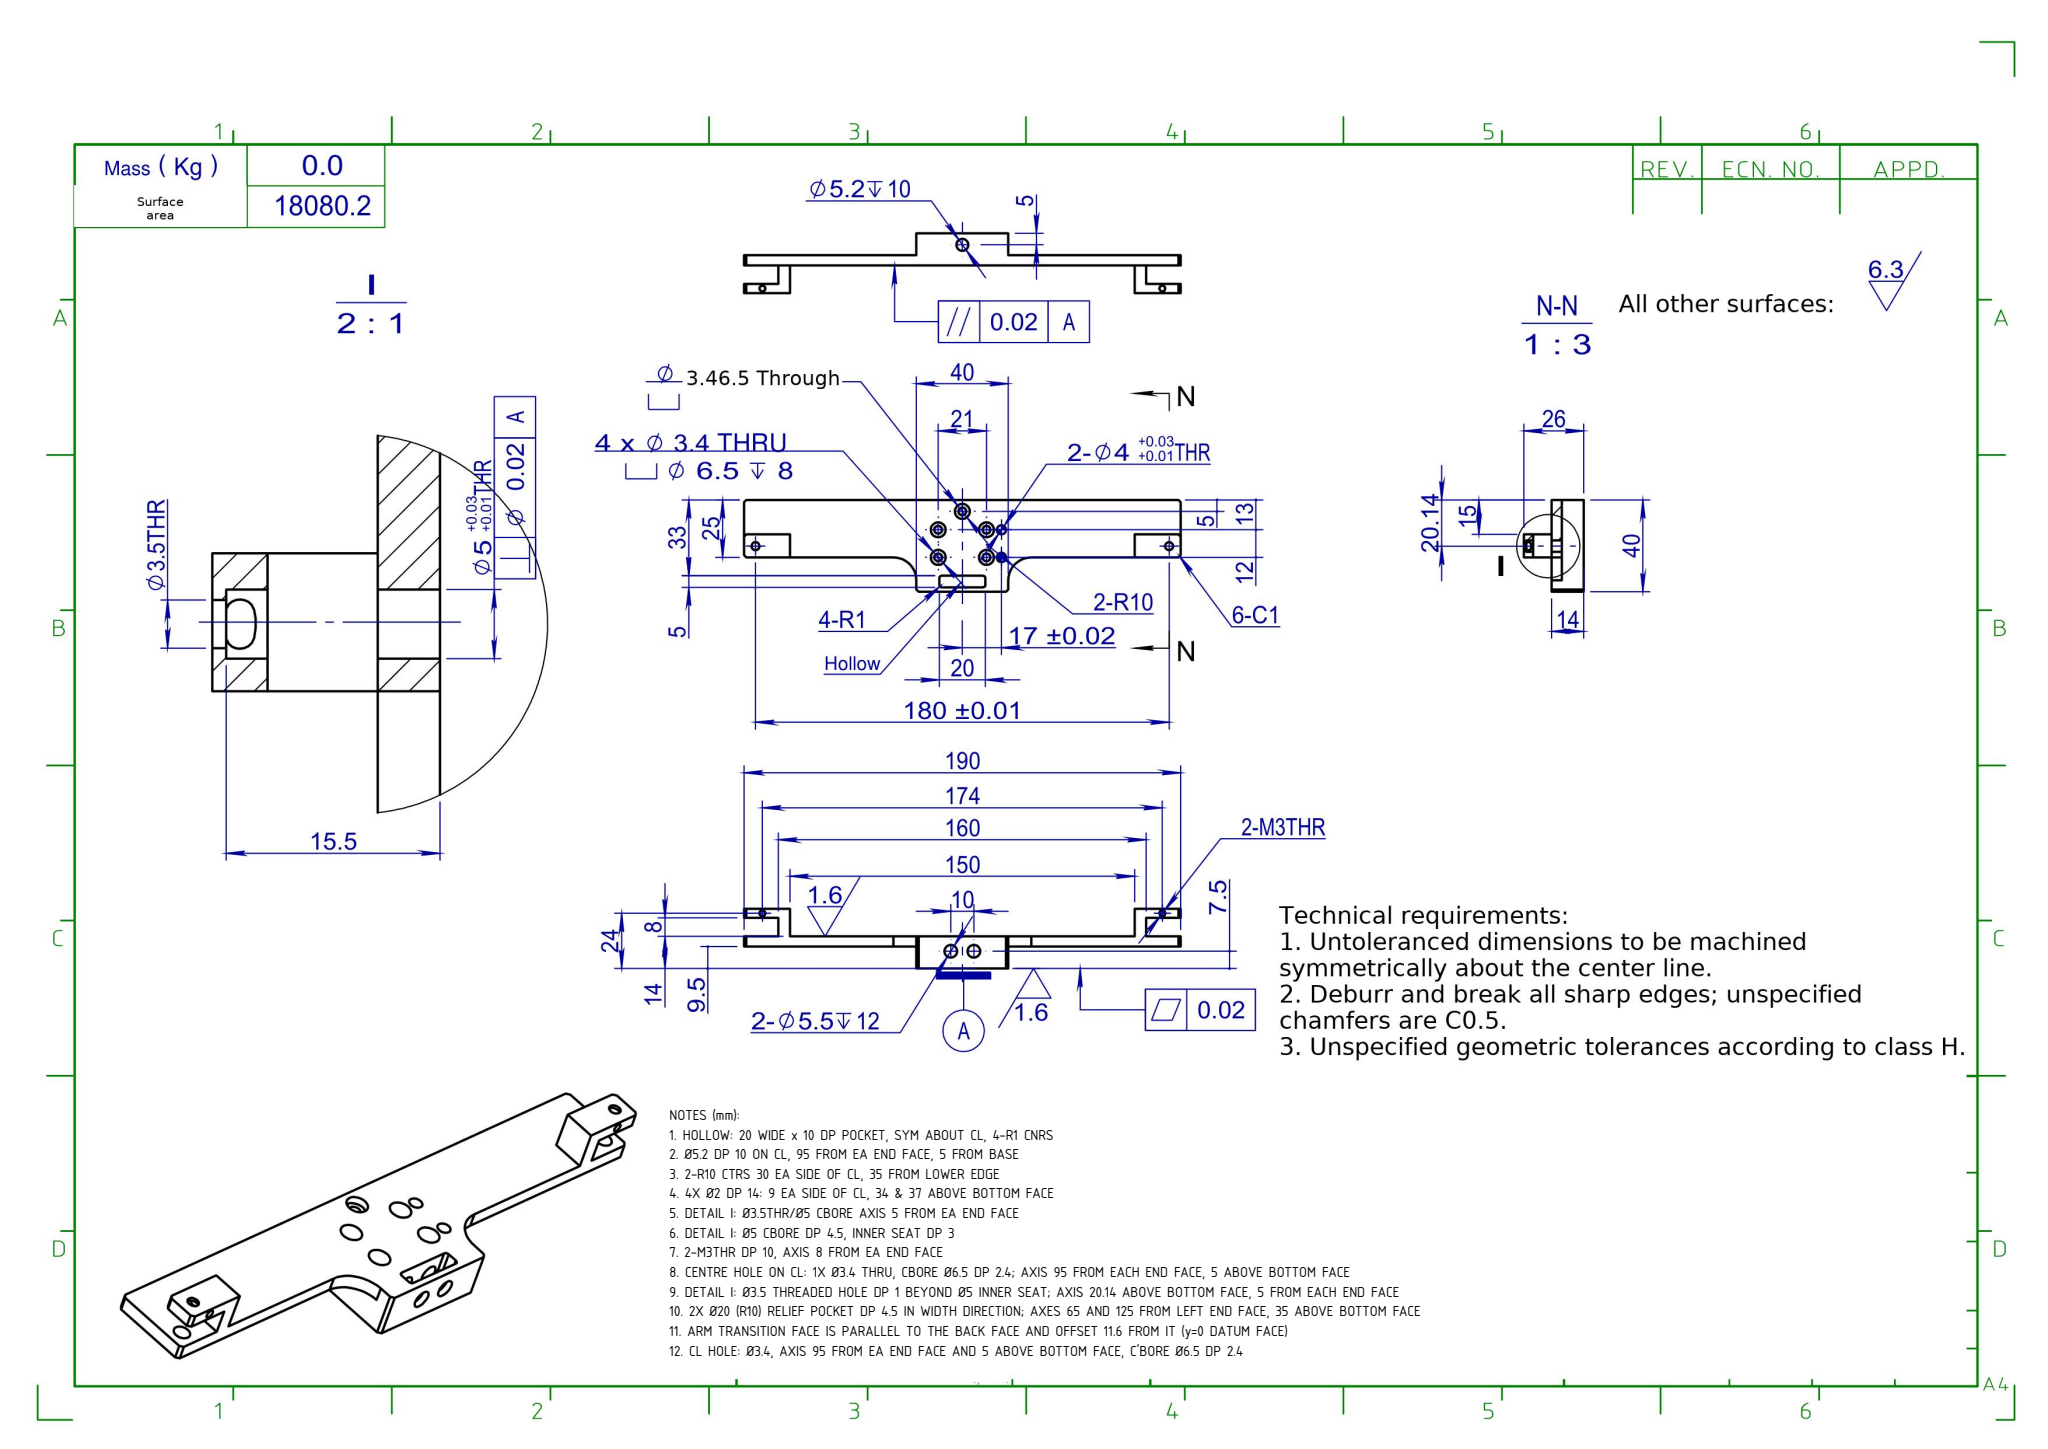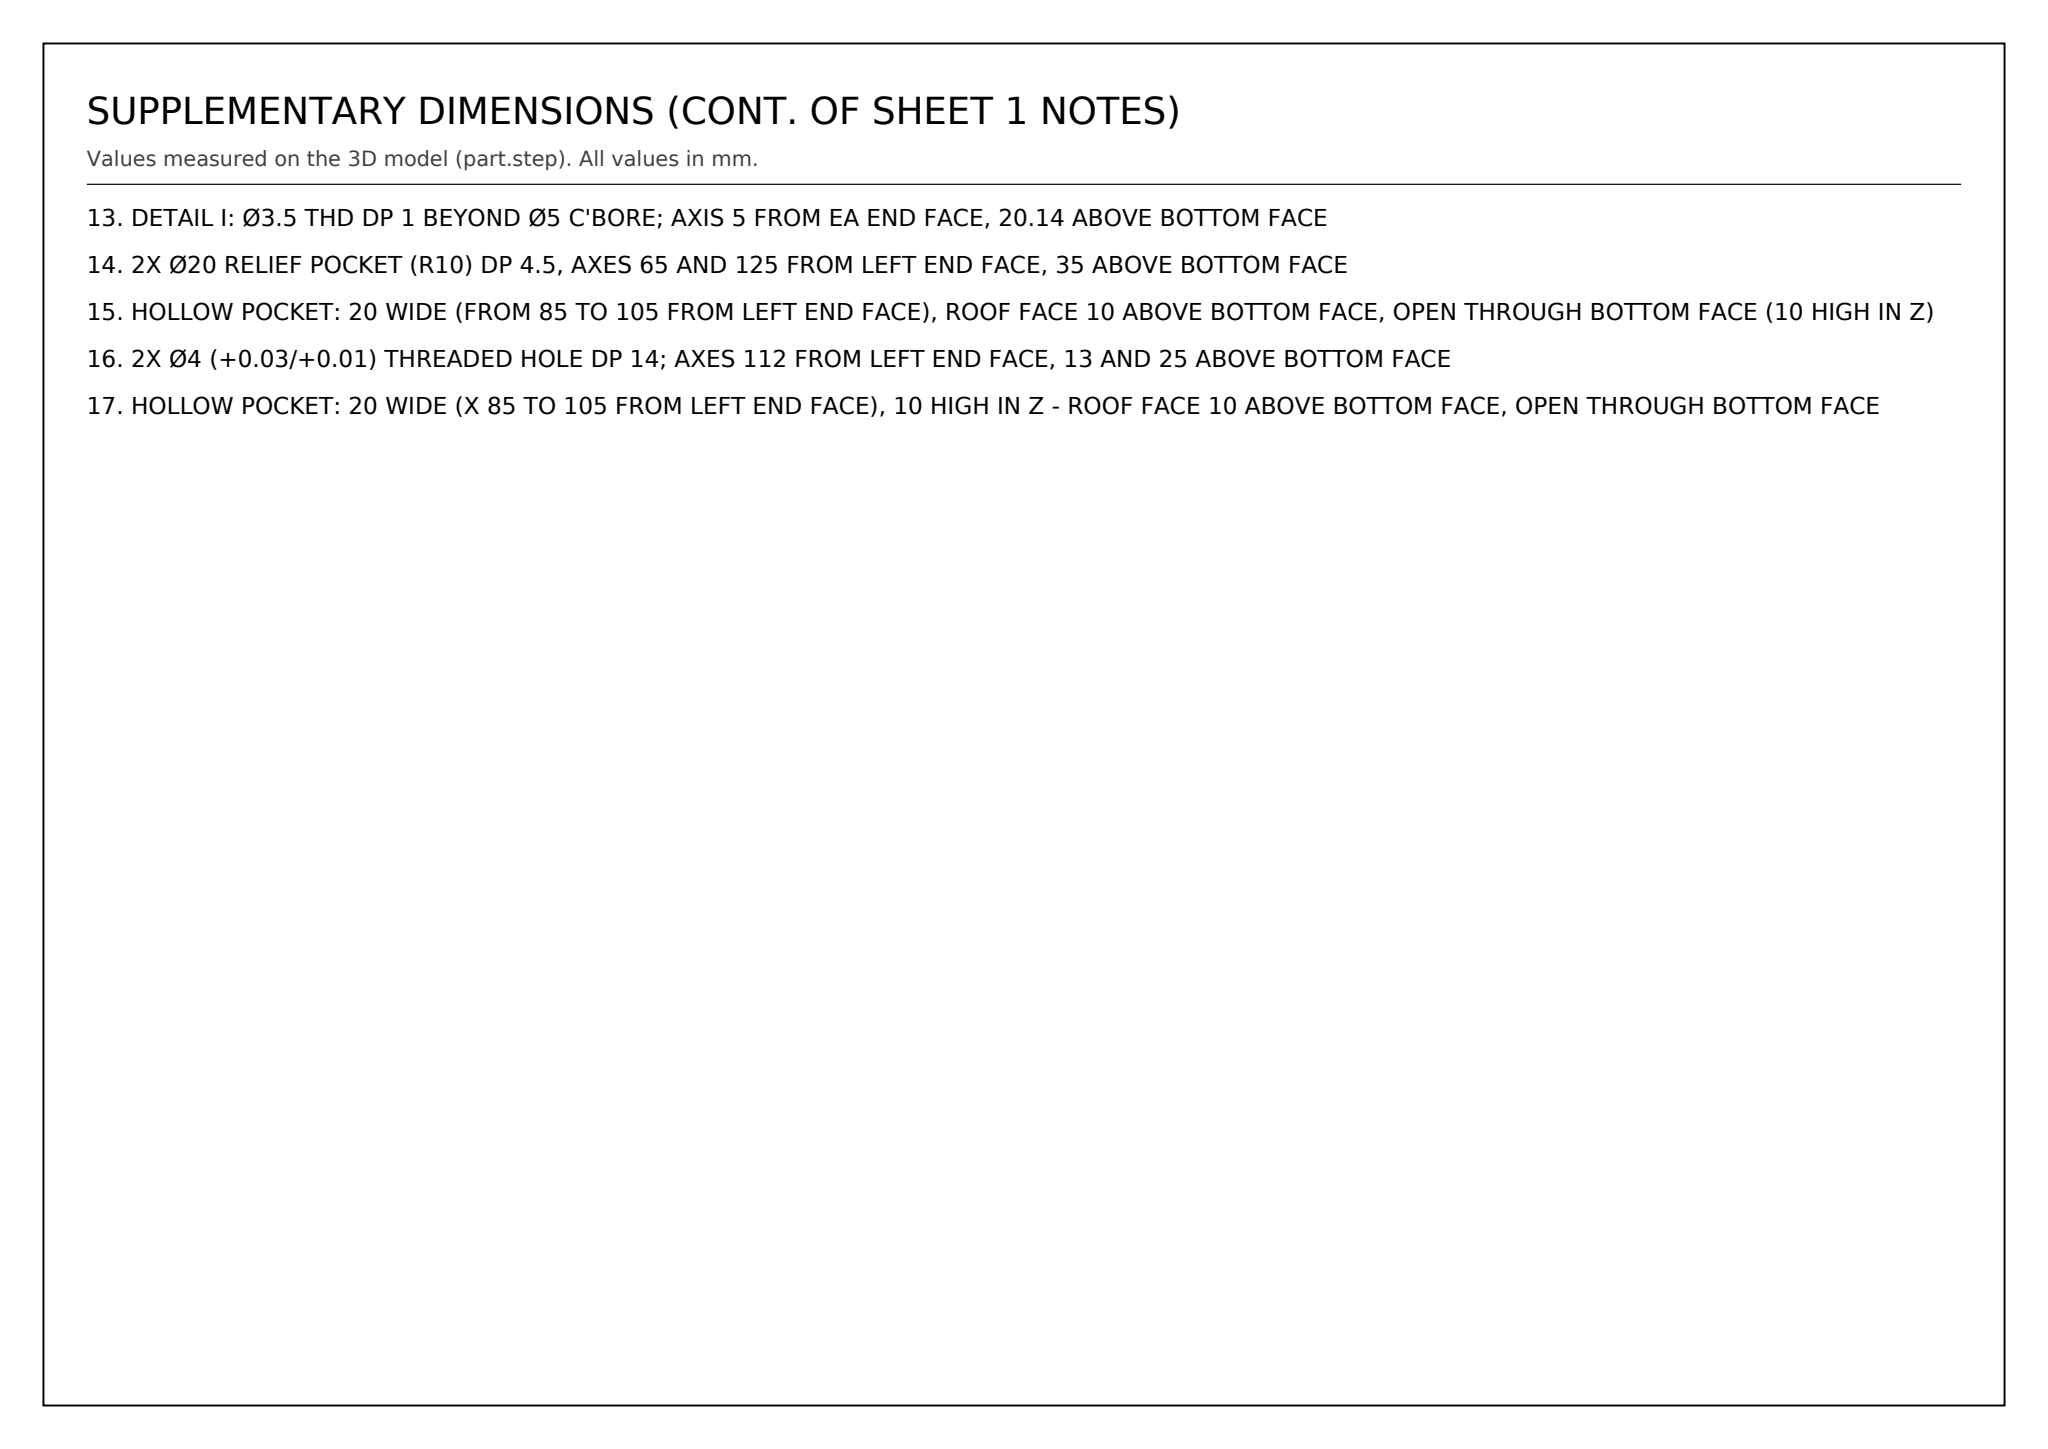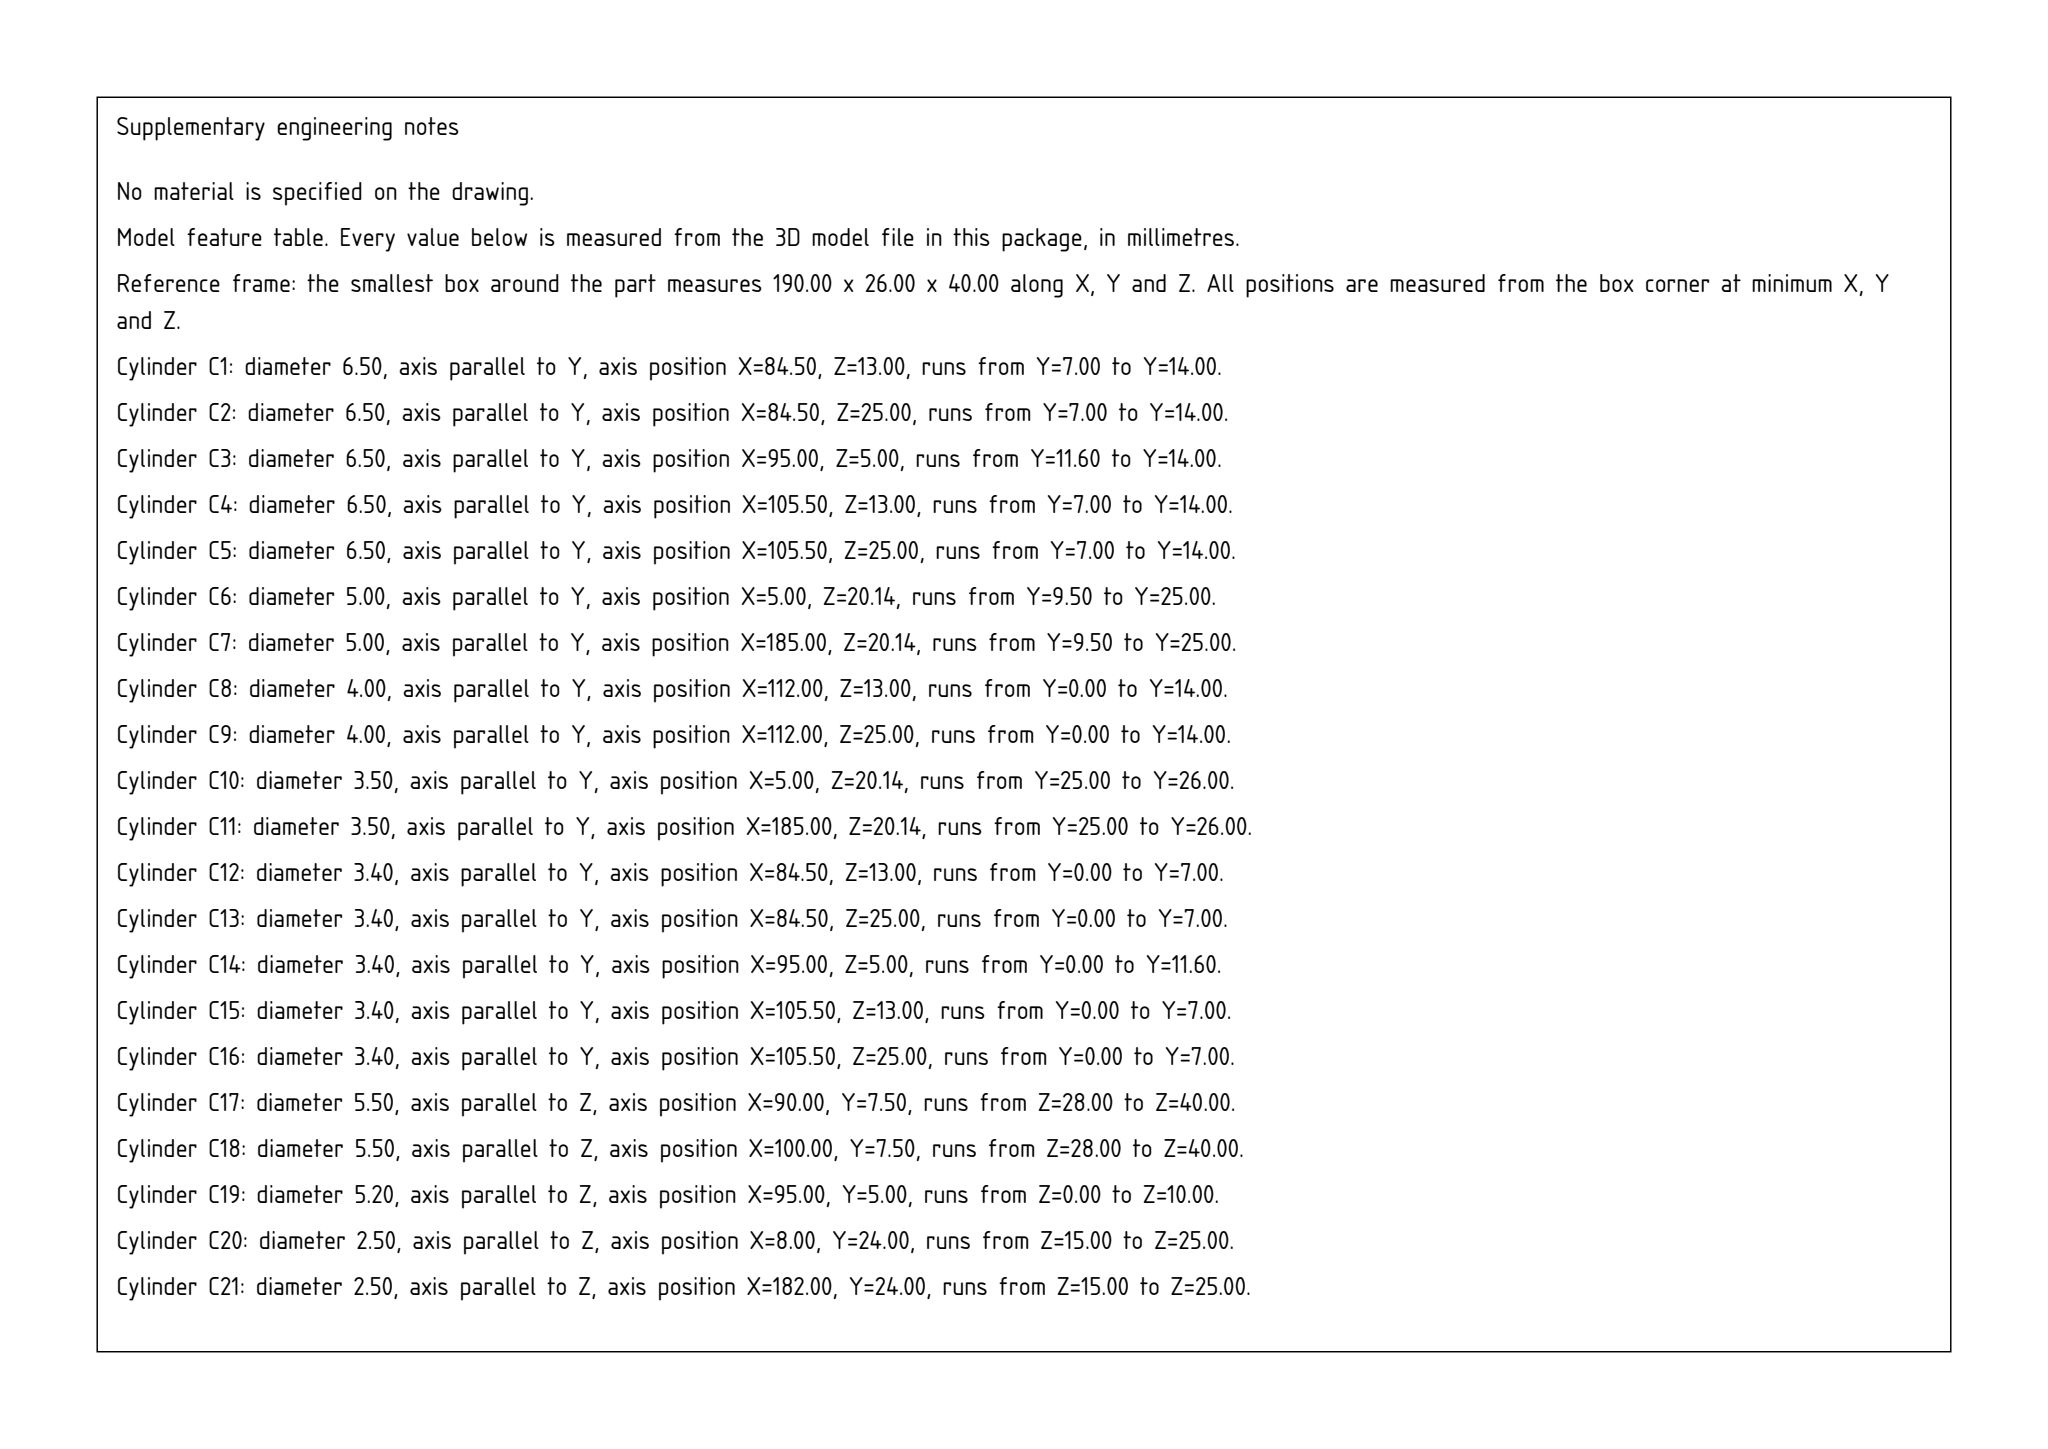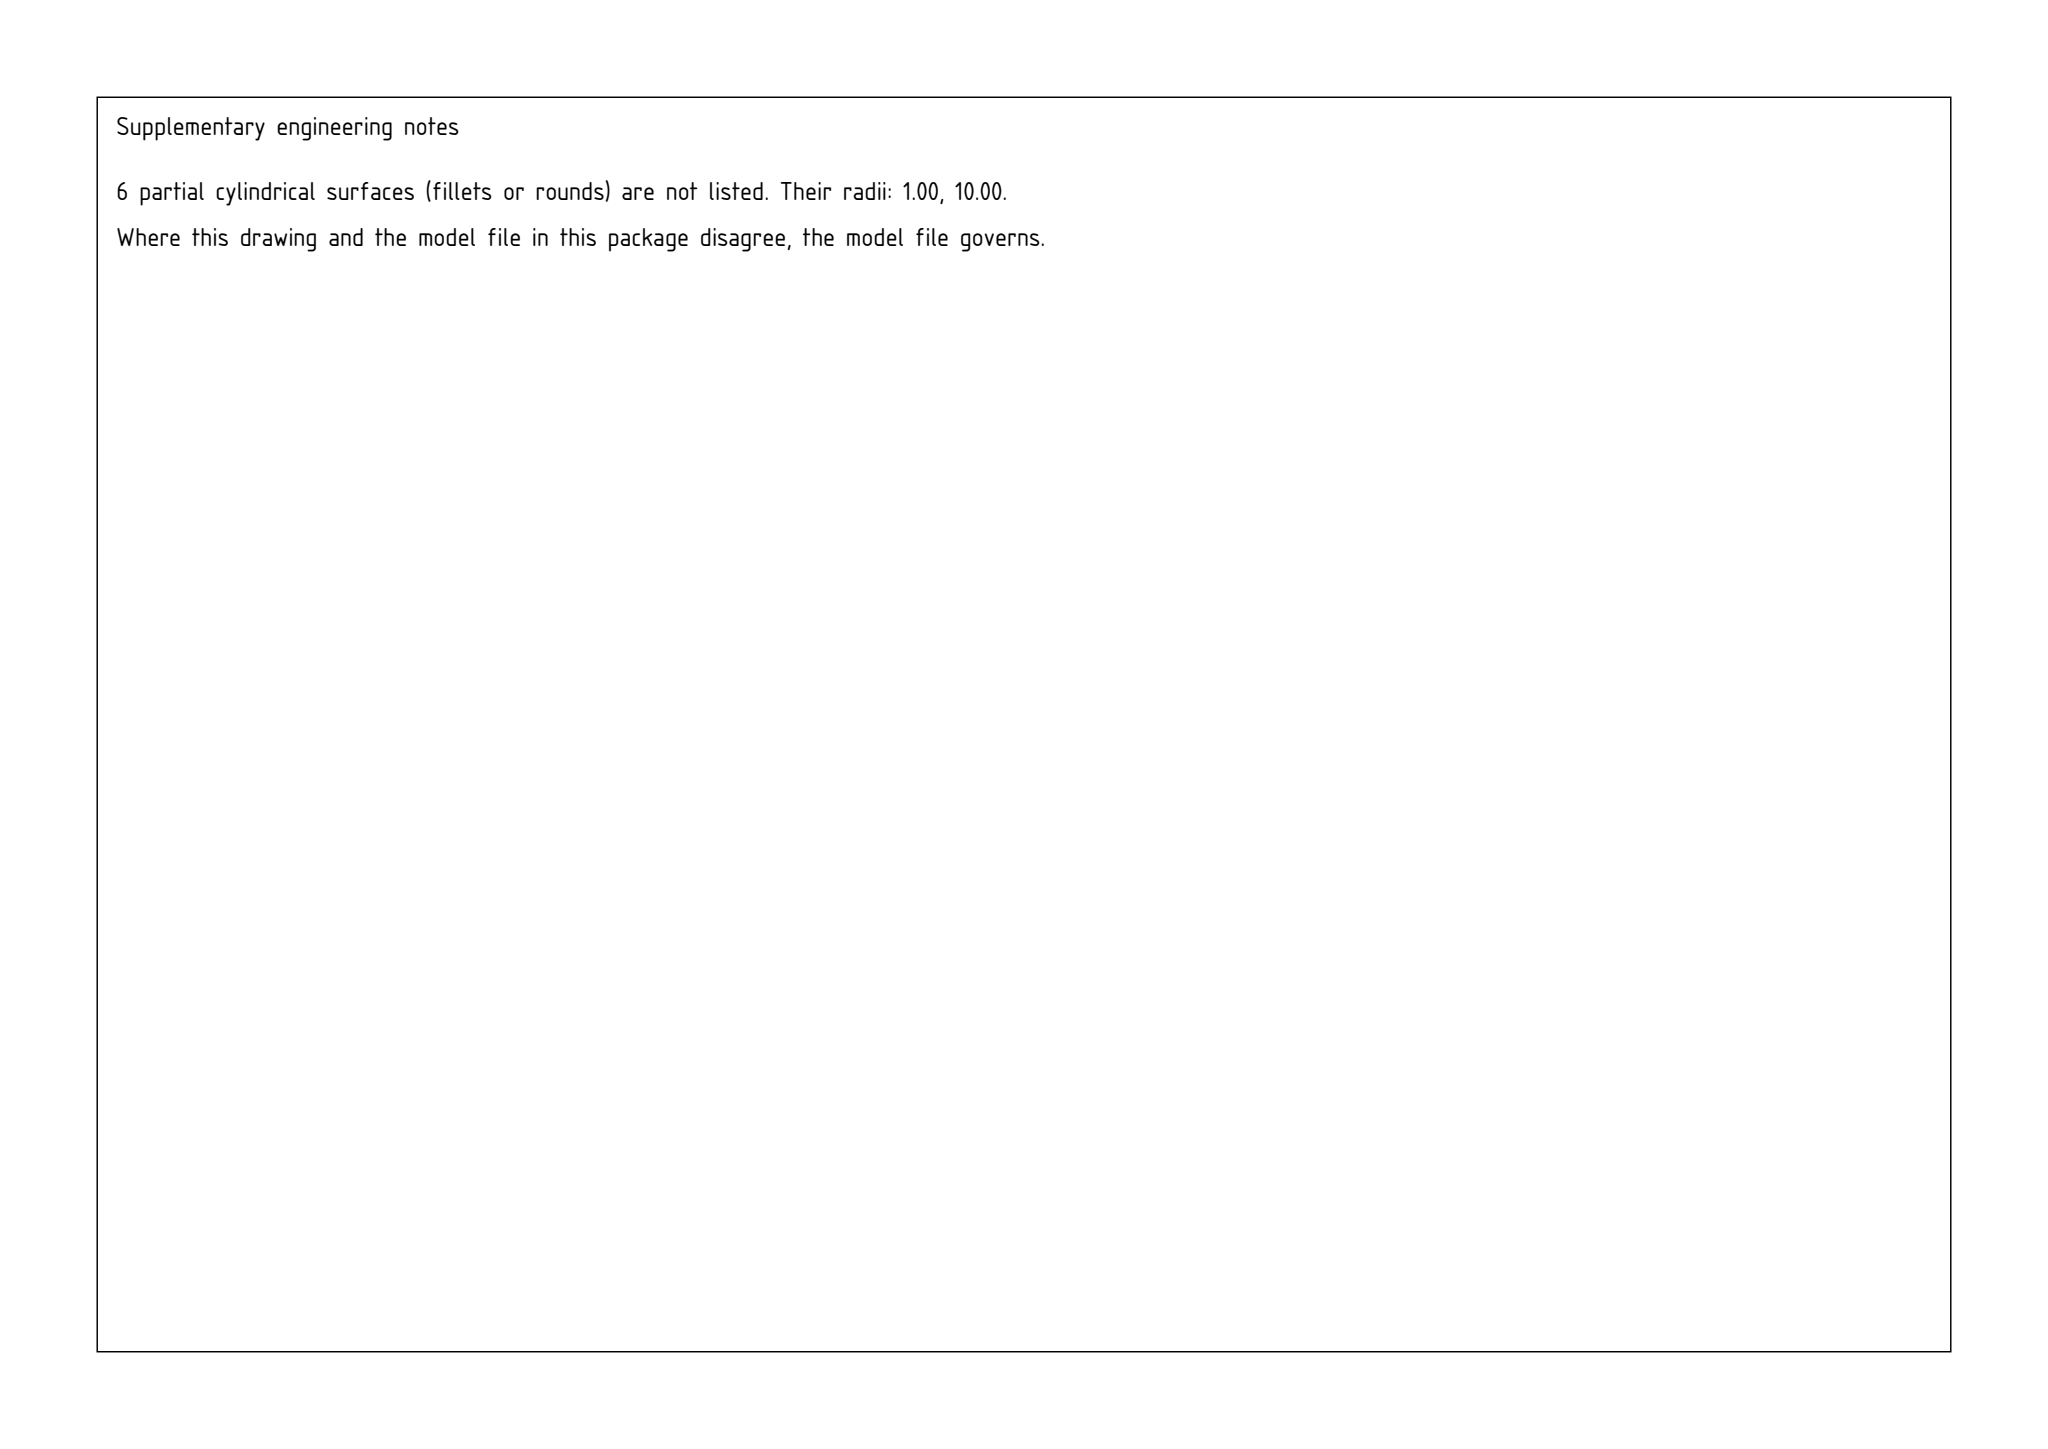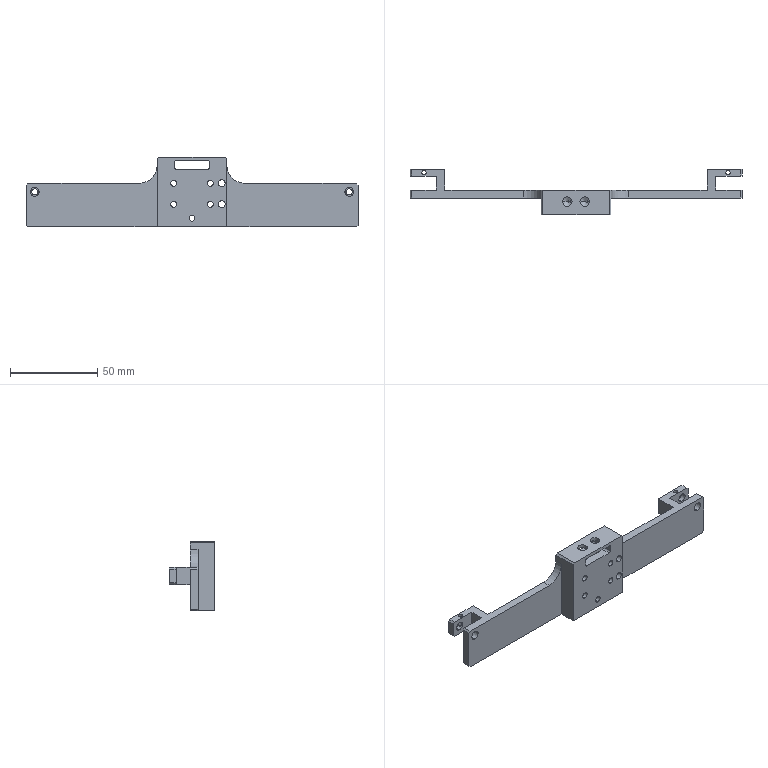Part | SolidWorks | mm | 1 solid | 108 faces | box 190 x 26 x 40 mm | volume 37796 mm3 | cylinder 58 | plane 46 | cone 4 | commonest cylinder face diameters 3.4 x12 6.5 x10 5 x8 5.5 x8 2.5 x4 3.5 x4 4 x4 2 x4
Drawing notes:
HOLLOW: 20 WIDE x 10 DP POCKET, SYM ABOUT CL, 4-R1 CNRS | from the solid: Bounding faces x=85 & x=105 (20 wide, sym about CL x=95 of 190 bbox); pocket floor z=10
Ø5.2 DP 10 ON CL, 95 FROM EA END FACE, 5 FROM BASE | from the solid: Cylinder [5.2,'z',[95.0,5.0],len 10]; bbox x=190 so x=95 is CL; y=5 from y0 face
2-R10 CTRS 30 EA SIDE OF CL, 35 FROM LOWER EDGE | from the solid: Cylinders [20.0,'y',[65.0,35.0],4.5] and [20.0,'y',[125.0,35.0],4.5]; CL x=95, tangent to x=75/x=115 and z=25
4X Ø2 DP 14: 9 EA SIDE OF CL, 34 & 37 ABOVE BOTTOM FACE | from the solid: Ø2.0 y-axis cyls at x=86 & 104 (CL x=95), z=34 & 37, len 14
DETAIL I: Ø3.5THR/Ø5 CBORE AXIS 5 FROM EA END FACE | from the solid: Ø3.5 & Ø5 y-axis cyls at x=5.0 and x=185.0, bbox x=190 (180±0.01 apart)
DETAIL I: Ø5 CBORE DP 4.5, INNER SEAT DP 3 | from the solid: Ø5.0 y-axis cyls at [5,20.14] & [185,20.14] with lengths 4.5 and 3.0
2-M3THR DP 10, AXIS 8 FROM EA END FACE | from the solid: Ø2.5 z-axis cyls at x=8.0 and x=182.0, y=24, length 10
CENTRE HOLE ON CL: 1X Ø3.4 THRU, CBORE Ø6.5 DP 2.4; AXIS 95 FROM EACH END FACE, 5 ABOVE BOTTOM FACE | from the solid: cylinders [3.4,'y',[95,null,5],...] and [6.5,'y',[95,null,5],2.4]
DETAIL I: Ø3.5 THREADED HOLE DP 1 BEYOND Ø5 INNER SEAT; AXIS 20.14 ABOVE BOTTOM FACE, 5 FROM EACH END FACE | from the solid: cylinders [3.5,'y',[5,null,20.14],1.0] and [3.5,'y',[185,null,20.14],1.0]
2X Ø20 (R10) RELIEF POCKET DP 4.5 IN WIDTH DIRECTION; AXES 65 AND 125 FROM LEFT END FACE, 35 ABOVE BOTTOM FACE | from the solid: cylinders [20.0,'y',[65,null,35],4.5] and [20.0,'y',[125,null,35],4.5]
ARM TRANSITION FACE IS PARALLEL TO THE BACK FACE AND OFFSET 11.6 FROM IT (y=0 DATUM FACE) | from the solid: axis_planes ['y',11.6]
CL HOLE: Ø3.4, AXIS 95 FROM EA END FACE AND 5 ABOVE BOTTOM FACE, C'BORE Ø6.5 DP 2.4 | from the solid: cylinders: [3.4,"y",[95,null,5],4.63] and [6.5,"y",[95,null,5],2.4]
DETAIL I: Ø3.5 THD DP 1 BEYOND Ø5 C'BORE; AXIS 5 FROM EA END FACE, 20.14 ABOVE BOTTOM FACE | from the solid: cylinders: [3.5,"y",[5,null,20.14],1.0] and [3.5,"y",[185,null,20.14],1.0]
2X Ø20 RELIEF POCKET (R10) DP 4.5, AXES 65 AND 125 FROM LEFT END FACE, 35 ABOVE BOTTOM FACE | from the solid: cylinders: [20,"y",[65,null,35],4.5] and [20,"y",[125,null,35],4.5]
HOLLOW POCKET: 20 WIDE (FROM 85 TO 105 FROM LEFT END FACE), ROOF FACE 10 ABOVE BOTTOM FACE, OPEN THROUGH BOTTOM FACE (10 HIGH IN Z) | from the solid: axis_planes x=85 and x=105 (20 apart), axis_plane z=10 (single horizontal roof face), z=0 bottom face
2X Ø4 (+0.03/+0.01) THREADED HOLE DP 14; AXES 112 FROM LEFT END FACE, 13 AND 25 ABOVE BOTTOM FACE | from the solid: cylinders [4.0,"y",[112.0,null,13.0],14.0] and [4.0,"y",[112.0,null,25.0],14.0]
HOLLOW POCKET: 20 WIDE (X 85 TO 105 FROM LEFT END FACE), 10 HIGH IN Z - ROOF FACE 10 ABOVE BOTTOM FACE, OPEN THROUGH BOTTOM FACE | from the solid: axis_planes x=85 and x=105 (20 apart), z=10 roof plane and z=0 bottom face
build123d program:
from build123d import *

# Parameters (mm, degrees)
SKETCH1_W                                           = 60
SKETCH1_H                                           = 40
EXTRUDE1_DEPTH                                      = 15
SKETCH6_W                                           = 10
SKETCH6_H                                           = 15
CUT_EXTRUDE3_DEPTH                                  = 40.051
SKETCH7_R                                           = 2.6
CUT_EXTRUDE4_DEPTH                                  = 10
COUNTERBORE_HOLE_FOR_M3_HEX_SOCKET_HEAD_D           = 3.4
COUNTERBORE_HOLE_FOR_M3_HEX_SOCKET_HEAD_CBORE_D     = 6.5
COUNTERBORE_HOLE_FOR_M3_HEX_SOCKET_HEAD_CBORE_DEPTH = 3.4
SKETCH13_W                                          = 10
SKETCH13_H                                          = 25
BOSS_EXTRUDE1_DEPTH                                 = 15
COUNTERBORE_HOLE_FOR_M3_HEX_SOCKET_H_2_D            = 3.4
COUNTERBORE_HOLE_FOR_M3_HEX_SOCKET_H_2_CBORE_D      = 6.5
COUNTERBORE_HOLE_FOR_M3_HEX_SOCKET_H_2_CBORE_DEPTH  = 8
SKETCH15_R                                          = 2
CUT_EXTRUDE7_DEPTH                                  = 48.17
SKETCH34_W                                          = 20
SKETCH34_H                                          = 9.5
CUT_EXTRUDE8_DEPTH                                  = 59.523
SKETCH35_W                                          = 55
SKETCH35_H                                          = 25
BOSS_EXTRUDE2_DEPTH                                 = 5.5
SKETCH37_R                                          = 2.5
CUT_EXTRUDE9_DEPTH                                  = 99.234
CUT_EXTRUDE11_DEPTH                                 = 1
SKETCH40_W                                          = 5
SKETCH40_H                                          = 10
BOSS_EXTRUDE4_DEPTH                                 = 12
M5_CLEARANCE_HOLE1_D                                = 5.5
M5_CLEARANCE_HOLE1_DEPTH                            = 12
M5_CLEARANCE_HOLE1_TIP                              = 1.652
SKETCH50_W                                          = 20
SKETCH50_H                                          = 5
CUT_EXTRUDE14_DEPTH                                 = 101.504
FILLET2_R                                           = 1
SKETCH51_W                                          = 15
SKETCH51_H                                          = 10
BOSS_EXTRUDE5_DEPTH                                 = 4
CUT_EXTRUDE15_START                                 = -3
SKETCH52_R                                          = 2.5
CUT_EXTRUDE15_DEPTH                                 = 3
SKETCH53_R                                          = 1.75
CUT_EXTRUDE16_DEPTH                                 = 101.25
FILLET3_R                                           = 10
CHAMFER1_SIZE                                       = 1
M3_THREADED_HOLE1_D                                 = 2.5


with BuildPart() as part:
    # Sketch1 → Extrude1 (new body)
    with BuildSketch(Plane(origin=(0, 0, 0), x_dir=(1, 0, 0), z_dir=(0, 1, 0))):
        Rectangle(SKETCH1_W, SKETCH1_H)
    extrude(amount=EXTRUDE1_DEPTH)

    # Sketch6 → Cut-Extrude3 (cut, through all)
    with BuildSketch(Plane(origin=(0, 15, 0), x_dir=(1, 0, 0), z_dir=(0, 1, 0))):
        with Locations((-25, -12.5)):
            Rectangle(SKETCH6_W, SKETCH6_H)
        with Locations((25, -12.5)):
            Rectangle(SKETCH6_W, SKETCH6_H)
    extrude(amount=-CUT_EXTRUDE3_DEPTH, mode=Mode.SUBTRACT)

    # Sketch7 → Cut-Extrude4 (cut)
    with BuildSketch(Plane(origin=(0, 0, -20), x_dir=(-1, 0, 0), z_dir=(0, 0, -1))):
        with Locations((0, 5)):
            Circle(SKETCH7_R)
    extrude(amount=-CUT_EXTRUDE4_DEPTH, mode=Mode.SUBTRACT)

    # Counterbore Hole for M3 Hex Socket Head (through all)
    with Locations(Plane(origin=(1.551, 15, -18.094), x_dir=(1, 0, 0), z_dir=(0, 1, 0))):
        with Locations((-1.551, -3.094)):
            CounterBoreHole(COUNTERBORE_HOLE_FOR_M3_HEX_SOCKET_HEAD_D / 2, COUNTERBORE_HOLE_FOR_M3_HEX_SOCKET_HEAD_CBORE_D / 2, COUNTERBORE_HOLE_FOR_M3_HEX_SOCKET_HEAD_CBORE_DEPTH)

    # Sketch13 → Boss-Extrude1 (add)
    with BuildSketch(Plane(origin=(0, 15, 0), x_dir=(1, 0, 0), z_dir=(0, 1, 0))):
        with Locations((-35, 7.5)):
            Rectangle(SKETCH13_W, SKETCH13_H)
        with Locations((35, 7.5)):
            Rectangle(SKETCH13_W, SKETCH13_H)
    extrude(amount=-BOSS_EXTRUDE1_DEPTH)

    # Counterbore Hole for M3 Hex Socket H 2 (through all)
    with Locations(Plane(origin=(0, 15, 0), x_dir=(-1, 0, 0), z_dir=(0, 1, 0))):
        with Locations((-10.5, -7), (10.5, -7), (-10.5, 5), (10.5, 5)):
            CounterBoreHole(COUNTERBORE_HOLE_FOR_M3_HEX_SOCKET_H_2_D / 2, COUNTERBORE_HOLE_FOR_M3_HEX_SOCKET_H_2_CBORE_D / 2, COUNTERBORE_HOLE_FOR_M3_HEX_SOCKET_H_2_CBORE_DEPTH)

    # Sketch15 → Cut-Extrude7 (cut, through all)
    with BuildSketch(Plane.XZ):
        with Locations(Location((17, 5, 0), (0, 0, 90))):
            Circle(SKETCH15_R)
        with Locations(Location((17, -7, 0), (0, 0, 90))):
            Circle(SKETCH15_R)
    extrude(amount=-CUT_EXTRUDE7_DEPTH, mode=Mode.SUBTRACT)

    # Sketch34 → Cut-Extrude8 (cut, through all)
    with BuildSketch(Plane(origin=(0, 0, -20), x_dir=(-1, 0, 0), z_dir=(0, 0, -1))):
        with Locations((-30, 4.75)):
            Rectangle(SKETCH34_W, SKETCH34_H)
        with Locations((30, 4.75)):
            Rectangle(SKETCH34_W, SKETCH34_H)
    extrude(amount=-CUT_EXTRUDE8_DEPTH, mode=Mode.SUBTRACT)

    # Sketch35 → Boss-Extrude2 (add)
    with BuildSketch(Plane.XZ.offset(-9.5)):
        with Locations((67.5, -7.5)):
            Rectangle(SKETCH35_W, SKETCH35_H)
        with Locations((-67.5, -7.5)):
            Rectangle(SKETCH35_W, SKETCH35_H)
    extrude(amount=-BOSS_EXTRUDE2_DEPTH)

    # Sketch37 → Cut-Extrude9 (cut, through all)
    with BuildSketch(Plane(origin=(0, 15, 0), x_dir=(1, 0, 0), z_dir=(0, 1, 0))):
        with Locations(Location((90, -0.135, 0), (0, 0, 270))):
            Circle(SKETCH37_R)
        with Locations(Location((-90, -0.135, 0), (0, 0, 270))):
            Circle(SKETCH37_R)
    extrude(amount=-CUT_EXTRUDE9_DEPTH, mode=Mode.SUBTRACT)

    # Sketch39 → Cut-Extrude11 (cut)
    with BuildSketch(Plane(origin=(0, 15, 0), x_dir=(1, 0, 0), z_dir=(0, 1, 0))):
        Polygon((95, 20), (-95, 20), (-95, -5), (-20, -5), (-20, -20), (20, -20), (20, -5), (95, -5), align=None)
    extrude(amount=-CUT_EXTRUDE11_DEPTH, mode=Mode.SUBTRACT)

    # Sketch40 → Boss-Extrude4 (add)
    with BuildSketch(Plane(origin=(0, 14, 0), x_dir=(1, 0, 0), z_dir=(0, 1, 0))):
        with Locations((77.5, 0)):
            Rectangle(SKETCH40_W, SKETCH40_H)
        with Locations((-77.5, 0)):
            Rectangle(SKETCH40_W, SKETCH40_H)
    extrude(amount=BOSS_EXTRUDE4_DEPTH)

    # M5 Clearance Hole1
    with Locations(Plane.XY.offset(20)):
        with Locations((-5, 7.5), (5, 7.5)):
            Hole(M5_CLEARANCE_HOLE1_D / 2, depth=M5_CLEARANCE_HOLE1_DEPTH)
            with Locations((0, 0, -(M5_CLEARANCE_HOLE1_DEPTH + M5_CLEARANCE_HOLE1_TIP / 2))):  # 118° drill point
                Cone(0, M5_CLEARANCE_HOLE1_D / 2, M5_CLEARANCE_HOLE1_TIP, mode=Mode.SUBTRACT)

    # Sketch50 → Cut-Extrude14 (cut, through all)
    with BuildSketch(Plane.XZ):
        with Locations((0, 15.5)):
            Rectangle(SKETCH50_W, SKETCH50_H)
    extrude(amount=-CUT_EXTRUDE14_DEPTH, mode=Mode.SUBTRACT)

    # Fillet2
    fillet2_edges = [part.edges().sort_by_distance(p)[0] for p in [
        (-10, 7, 18),
        (10, 7, 13),
        (-10, 7, 13),
        (10, 7, 18),
    ]]
    fillet(fillet2_edges, radius=FILLET2_R)

    # Sketch51 → Boss-Extrude5 (add)
    with BuildSketch(Plane(origin=(0, 26, 0), x_dir=(1, 0, 0), z_dir=(0, 1, 0))):
        with Locations((-87.5, 0)):
            Rectangle(SKETCH51_W, SKETCH51_H)
        with Locations((87.5, 0)):
            Rectangle(SKETCH51_W, SKETCH51_H)
    extrude(amount=-BOSS_EXTRUDE5_DEPTH)

    # Sketch52 → Cut-Extrude15 (cut)
    with BuildSketch(Plane.XZ.offset(-22).offset(CUT_EXTRUDE15_START)):
        with Locations(Location((90, 0.135, 0), (0, 0, 90))):
            Circle(SKETCH52_R)
        with Locations(Location((-90, 0.135, 0), (0, 0, 90))):
            Circle(SKETCH52_R)
    extrude(amount=CUT_EXTRUDE15_DEPTH, mode=Mode.SUBTRACT)

    # Sketch53 → Cut-Extrude16 (cut, through all)
    with BuildSketch(Plane.XZ.offset(-25)):
        with Locations(Location((-90, 0.135, 0), (0, 0, 270))):
            Circle(SKETCH53_R)
        with Locations(Location((90, 0.135, 0), (0, 0, 270))):
            Circle(SKETCH53_R)
    extrude(amount=-CUT_EXTRUDE16_DEPTH, mode=Mode.SUBTRACT)

    # Fillet3
    fillet3_edges = [part.edges().sort_by_distance(p)[0] for p in [
        (20, 11.75, 5),
        (-20, 11.75, 5),
    ]]
    fillet(fillet3_edges, radius=FILLET3_R)

    # Chamfer1
    chamfer1_edges = [part.edges().sort_by_distance(p)[0] for p in [
        (-20, 7, 20),
        (-95, 11.75, 5),
        (-95, 11.75, -20),
        (95, 11.75, -20),
        (95, 11.75, 5),
        (20, 7, 20),
        (-95, 24, 5),
        (-95, 24, -5),
        (95, 24, -5),
        (95, 24, 5),
    ]]
    chamfer(chamfer1_edges, length=CHAMFER1_SIZE)

    # M3 Threaded Hole1 (through all)
    with Locations(Plane.XY.offset(5)):
        with Locations((-87, 24)):
            m3_threaded_hole1 = Hole(M3_THREADED_HOLE1_D / 2)

    # Mirror1: M3 Threaded Hole1 across plane
    add(m3_threaded_hole1.mirror(Plane(origin=(0, 0, 0), x_dir=(0, 0, 1), z_dir=(1, 0, 0))), mode=Mode.SUBTRACT)


solid = part.part